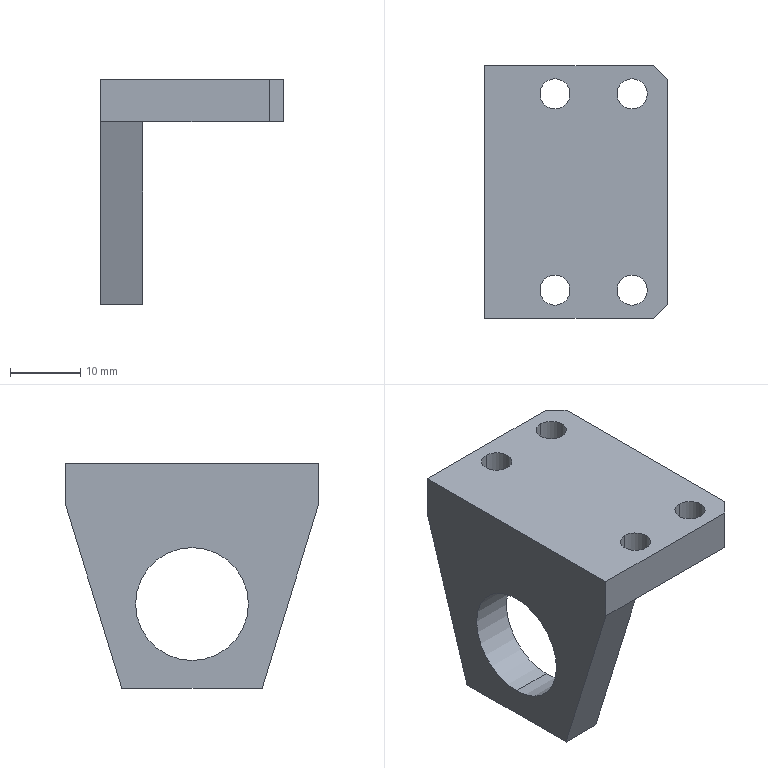Component | SolidWorks | 05-1111-1 | 1 solid | 22 faces | box 26 x 36 x 32 mm | volume 8390 mm3 | plane 12 | cylinder 10 | commonest cylinder face diameters 4.3 x8 16.1 x2 | material Plain Carbon Steel
build123d program:
from build123d import *

# Parameters (mm, degrees)
BOSS_EXTRUDE1_DEPTH        = 18
SKETCH2_R                  = 8.05
CUT_EXTRUDE1_DEPTH         = 42.809
F_4_3_4_3_DIAMETER_HOLE1_D = 4.3
CHAMFER1_SIZE              = 2
CUT_EXTRUDE4_DEPTH         = 41.939


with BuildPart() as part:
    # Sketch1 → Boss-Extrude1 (new, symmetric)
    with BuildSketch(Plane.XY):
        Polygon((0, 0), (32, 0), (32, 6), (6, 6), (6, 26), (0, 26), align=None)
    extrude(amount=BOSS_EXTRUDE1_DEPTH, both=True)

    # Sketch2 → Cut-Extrude1 (cut, through all)
    with BuildSketch(Plane(origin=(0, 6, 0), x_dir=(1, 0, 0), z_dir=(0, 1, 0))):
        with Locations(Location((20, 0, 0), (0, 0, 180))):
            Circle(SKETCH2_R)
    extrude(amount=-CUT_EXTRUDE1_DEPTH, mode=Mode.SUBTRACT)

    # 4.3 _4.3_ Diameter Hole1 (through all)
    with Locations(Plane(origin=(6, 0, 0), x_dir=(0, 0, -1), z_dir=(1, 0, 0))):
        with Locations((-14, 21), (-14, 10), (14, 10), (14, 21)):
            Hole(F_4_3_4_3_DIAMETER_HOLE1_D / 2)

    # Chamfer1
    chamfer1_edges = [part.edges().sort_by_distance(p)[0] for p in [
        (3, 26, 18),
        (3, 26, -18),
    ]]
    chamfer(chamfer1_edges, length=CHAMFER1_SIZE)

    # Sketch5 → Cut-Extrude4 (cut, through all)
    with BuildSketch(Plane(origin=(6, 0, 0), x_dir=(0, 0, -1), z_dir=(0, 1, 0))):
        Polygon((-18, -26), (-10, -26), (-18, 0), align=None)
        Polygon((10, -26), (18, 0), (18, -26), align=None)
    extrude(amount=CUT_EXTRUDE4_DEPTH, mode=Mode.SUBTRACT)


solid = part.part

# Placed as in the assembly
solid = solid.moved(Location((-105, 24, -6), (90, 0, -90)))
STEP:
#1=CARTESIAN_POINT('',(-3.307,0.3091,-0.2362));
#2=VERTEX_POINT('',#1);
#3=CARTESIAN_POINT('',(-3.307,0.4783,-0.2362));
#4=VERTEX_POINT('',#3);
#5=CARTESIAN_POINT('',(-3.307,0.3937,-0.2362));
#6=DIRECTION('',(0.,0.,-1.));
#7=DIRECTION('',(0.,1.,0.));
#8=AXIS2_PLACEMENT_3D('',#5,#6,#7);
#9=CIRCLE('',#8,0.08465);
#10=EDGE_CURVE('',#2,#4,#9,.T.);
#11=ORIENTED_EDGE('',*,*,#10,.F.);
#12=CARTESIAN_POINT('',(-3.307,0.3091,-0.4724));
#13=VERTEX_POINT('',#12);
#14=CARTESIAN_POINT('',(-3.307,0.3091,-0.4724));
#15=DIRECTION('',(0.,0.,-1.));
#16=VECTOR('',#15,39.37);
#17=LINE('',#14,#16);
#18=EDGE_CURVE('',#2,#13,#17,.T.);
#19=ORIENTED_EDGE('',*,*,#18,.T.);
#20=CARTESIAN_POINT('',(-3.307,0.4783,-0.4724));
#21=VERTEX_POINT('',#20);
#22=CARTESIAN_POINT('',(-3.307,0.3937,-0.4724));
#23=DIRECTION('',(0.,0.,-1.));
#24=DIRECTION('',(0.,1.,0.));
#25=AXIS2_PLACEMENT_3D('',#22,#23,#24);
#26=CIRCLE('',#25,0.08465);
#27=EDGE_CURVE('',#13,#21,#26,.T.);
#28=ORIENTED_EDGE('',*,*,#27,.T.);
#29=CARTESIAN_POINT('',(-3.307,0.4783,-0.4724));
#30=DIRECTION('',(0.,0.,-1.));
#31=VECTOR('',#30,39.37);
#32=LINE('',#29,#31);
#33=EDGE_CURVE('',#4,#21,#32,.T.);
#34=ORIENTED_EDGE('',*,*,#33,.F.);
#35=EDGE_LOOP('',(#11,#19,#28,#34));
#36=FACE_OUTER_BOUND('',#35,.T.);
#37=CARTESIAN_POINT('',(-3.307,0.3937,-0.4724));
#38=DIRECTION('',(0.,0.,-1.));
#39=DIRECTION('',(0.,1.,0.));
#40=AXIS2_PLACEMENT_3D('',#37,#38,#39);
#41=CYLINDRICAL_SURFACE('',#40,0.08465);
#42=ADVANCED_FACE('',(#36),#41,.F.);
#43=CARTESIAN_POINT('',(-3.74,0.3091,-0.2362));
#44=VERTEX_POINT('',#43);
#45=CARTESIAN_POINT('',(-3.74,0.4783,-0.2362));
#46=VERTEX_POINT('',#45);
#47=CARTESIAN_POINT('',(-3.74,0.3937,-0.2362));
#48=DIRECTION('',(0.,0.,-1.));
#49=DIRECTION('',(0.,1.,0.));
#50=AXIS2_PLACEMENT_3D('',#47,#48,#49);
#51=CIRCLE('',#50,0.08465);
#52=EDGE_CURVE('',#44,#46,#51,.T.);
#53=ORIENTED_EDGE('',*,*,#52,.F.);
#54=CARTESIAN_POINT('',(-3.74,0.3091,-0.4724));
#55=VERTEX_POINT('',#54);
#56=CARTESIAN_POINT('',(-3.74,0.3091,-0.4724));
#57=DIRECTION('',(0.,0.,-1.));
#58=VECTOR('',#57,39.37);
#59=LINE('',#56,#58);
#60=EDGE_CURVE('',#44,#55,#59,.T.);
#61=ORIENTED_EDGE('',*,*,#60,.T.);
#62=CARTESIAN_POINT('',(-3.74,0.4783,-0.4724));
#63=VERTEX_POINT('',#62);
#64=CARTESIAN_POINT('',(-3.74,0.3937,-0.4724));
#65=DIRECTION('',(0.,0.,-1.));
#66=DIRECTION('',(0.,1.,0.));
#67=AXIS2_PLACEMENT_3D('',#64,#65,#66);
#68=CIRCLE('',#67,0.08465);
#69=EDGE_CURVE('',#55,#63,#68,.T.);
#70=ORIENTED_EDGE('',*,*,#69,.T.);
#71=CARTESIAN_POINT('',(-3.74,0.4783,-0.4724));
#72=DIRECTION('',(0.,0.,-1.));
#73=VECTOR('',#72,39.37);
#74=LINE('',#71,#73);
#75=EDGE_CURVE('',#46,#63,#74,.T.);
#76=ORIENTED_EDGE('',*,*,#75,.F.);
#77=EDGE_LOOP('',(#53,#61,#70,#76));
#78=FACE_OUTER_BOUND('',#77,.T.);
#79=CARTESIAN_POINT('',(-3.74,0.3937,-0.4724));
#80=DIRECTION('',(0.,0.,-1.));
#81=DIRECTION('',(0.,1.,0.));
#82=AXIS2_PLACEMENT_3D('',#79,#80,#81);
#83=CYLINDRICAL_SURFACE('',#82,0.08465);
#84=ADVANCED_FACE('',(#78),#83,.F.);
#85=CARTESIAN_POINT('',(-3.74,1.411,-0.2362));
#86=VERTEX_POINT('',#85);
#87=CARTESIAN_POINT('',(-3.74,1.581,-0.2362));
#88=VERTEX_POINT('',#87);
#89=CARTESIAN_POINT('',(-3.74,1.496,-0.2362));
#90=DIRECTION('',(0.,0.,-1.));
#91=DIRECTION('',(0.,1.,0.));
#92=AXIS2_PLACEMENT_3D('',#89,#90,#91);
#93=CIRCLE('',#92,0.08465);
#94=EDGE_CURVE('',#86,#88,#93,.T.);
#95=ORIENTED_EDGE('',*,*,#94,.F.);
#96=CARTESIAN_POINT('',(-3.74,1.411,-0.4724));
#97=VERTEX_POINT('',#96);
#98=CARTESIAN_POINT('',(-3.74,1.411,-0.4724));
#99=DIRECTION('',(0.,0.,-1.));
#100=VECTOR('',#99,39.37);
#101=LINE('',#98,#100);
#102=EDGE_CURVE('',#86,#97,#101,.T.);
#103=ORIENTED_EDGE('',*,*,#102,.T.);
#104=CARTESIAN_POINT('',(-3.74,1.581,-0.4724));
#105=VERTEX_POINT('',#104);
#106=CARTESIAN_POINT('',(-3.74,1.496,-0.4724));
#107=DIRECTION('',(0.,0.,-1.));
#108=DIRECTION('',(0.,1.,0.));
#109=AXIS2_PLACEMENT_3D('',#106,#107,#108);
#110=CIRCLE('',#109,0.08465);
#111=EDGE_CURVE('',#97,#105,#110,.T.);
#112=ORIENTED_EDGE('',*,*,#111,.T.);
#113=CARTESIAN_POINT('',(-3.74,1.581,-0.4724));
#114=DIRECTION('',(0.,0.,-1.));
#115=VECTOR('',#114,39.37);
#116=LINE('',#113,#115);
#117=EDGE_CURVE('',#88,#105,#116,.T.);
#118=ORIENTED_EDGE('',*,*,#117,.F.);
#119=EDGE_LOOP('',(#95,#103,#112,#118));
#120=FACE_OUTER_BOUND('',#119,.T.);
#121=CARTESIAN_POINT('',(-3.74,1.496,-0.4724));
#122=DIRECTION('',(0.,0.,-1.));
#123=DIRECTION('',(0.,1.,0.));
#124=AXIS2_PLACEMENT_3D('',#121,#122,#123);
#125=CYLINDRICAL_SURFACE('',#124,0.08465);
#126=ADVANCED_FACE('',(#120),#125,.F.);
#127=CARTESIAN_POINT('',(-3.307,1.411,-0.2362));
#128=VERTEX_POINT('',#127);
#129=CARTESIAN_POINT('',(-3.307,1.581,-0.2362));
#130=VERTEX_POINT('',#129);
#131=CARTESIAN_POINT('',(-3.307,1.496,-0.2362));
#132=DIRECTION('',(0.,0.,-1.));
#133=DIRECTION('',(0.,1.,0.));
#134=AXIS2_PLACEMENT_3D('',#131,#132,#133);
#135=CIRCLE('',#134,0.08465);
#136=EDGE_CURVE('',#128,#130,#135,.T.);
#137=ORIENTED_EDGE('',*,*,#136,.F.);
#138=CARTESIAN_POINT('',(-3.307,1.411,-0.4724));
#139=VERTEX_POINT('',#138);
#140=CARTESIAN_POINT('',(-3.307,1.411,-0.4724));
#141=DIRECTION('',(0.,0.,-1.));
#142=VECTOR('',#141,39.37);
#143=LINE('',#140,#142);
#144=EDGE_CURVE('',#128,#139,#143,.T.);
#145=ORIENTED_EDGE('',*,*,#144,.T.);
#146=CARTESIAN_POINT('',(-3.307,1.581,-0.4724));
#147=VERTEX_POINT('',#146);
#148=CARTESIAN_POINT('',(-3.307,1.496,-0.4724));
#149=DIRECTION('',(0.,0.,-1.));
#150=DIRECTION('',(0.,1.,0.));
#151=AXIS2_PLACEMENT_3D('',#148,#149,#150);
#152=CIRCLE('',#151,0.08465);
#153=EDGE_CURVE('',#139,#147,#152,.T.);
#154=ORIENTED_EDGE('',*,*,#153,.T.);
#155=CARTESIAN_POINT('',(-3.307,1.581,-0.4724));
#156=DIRECTION('',(0.,0.,-1.));
#157=VECTOR('',#156,39.37);
#158=LINE('',#155,#157);
#159=EDGE_CURVE('',#130,#147,#158,.T.);
#160=ORIENTED_EDGE('',*,*,#159,.F.);
#161=EDGE_LOOP('',(#137,#145,#154,#160));
#162=FACE_OUTER_BOUND('',#161,.T.);
#163=CARTESIAN_POINT('',(-3.307,1.496,-0.4724));
#164=DIRECTION('',(0.,0.,-1.));
#165=DIRECTION('',(0.,1.,0.));
#166=AXIS2_PLACEMENT_3D('',#163,#164,#165);
#167=CYLINDRICAL_SURFACE('',#166,0.08465);
#168=ADVANCED_FACE('',(#162),#167,.F.);
#169=CARTESIAN_POINT('',(-4.134,0.9449,-1.341));
#170=VERTEX_POINT('',#169);
#171=CARTESIAN_POINT('',(-4.134,0.9449,-0.7067));
#172=VERTEX_POINT('',#171);
#173=CARTESIAN_POINT('',(-4.134,0.9449,-1.024));
#174=DIRECTION('',(1.,0.,-0.));
#175=DIRECTION('',(0.,0.,1.));
#176=AXIS2_PLACEMENT_3D('',#173,#174,#175);
#177=CIRCLE('',#176,0.3169);
#178=EDGE_CURVE('',#170,#172,#177,.T.);
#179=ORIENTED_EDGE('',*,*,#178,.F.);
#180=CARTESIAN_POINT('',(-3.898,0.9449,-1.341));
#181=VERTEX_POINT('',#180);
#182=CARTESIAN_POINT('',(-4.134,0.9449,-1.341));
#183=DIRECTION('',(1.,0.,-0.));
#184=VECTOR('',#183,39.37);
#185=LINE('',#182,#184);
#186=EDGE_CURVE('',#170,#181,#185,.T.);
#187=ORIENTED_EDGE('',*,*,#186,.T.);
#188=CARTESIAN_POINT('',(-3.898,0.9449,-0.7067));
#189=VERTEX_POINT('',#188);
#190=CARTESIAN_POINT('',(-3.898,0.9449,-1.024));
#191=DIRECTION('',(1.,0.,-0.));
#192=DIRECTION('',(0.,0.,1.));
#193=AXIS2_PLACEMENT_3D('',#190,#191,#192);
#194=CIRCLE('',#193,0.3169);
#195=EDGE_CURVE('',#181,#189,#194,.T.);
#196=ORIENTED_EDGE('',*,*,#195,.T.);
#197=CARTESIAN_POINT('',(-4.134,0.9449,-0.7067));
#198=DIRECTION('',(1.,0.,-0.));
#199=VECTOR('',#198,39.37);
#200=LINE('',#197,#199);
#201=EDGE_CURVE('',#172,#189,#200,.T.);
#202=ORIENTED_EDGE('',*,*,#201,.F.);
#203=EDGE_LOOP('',(#179,#187,#196,#202));
#204=FACE_OUTER_BOUND('',#203,.T.);
#205=CARTESIAN_POINT('',(-4.134,0.9449,-1.024));
#206=DIRECTION('',(1.,0.,-0.));
#207=DIRECTION('',(0.,0.,1.));
#208=AXIS2_PLACEMENT_3D('',#205,#206,#207);
#209=CYLINDRICAL_SURFACE('',#208,0.3169);
#210=ADVANCED_FACE('',(#204),#209,.F.);
#211=CARTESIAN_POINT('',(-4.134,0.9449,-1.024));
#212=DIRECTION('',(1.,0.,-0.));
#213=DIRECTION('',(0.,0.,1.));
#214=AXIS2_PLACEMENT_3D('',#211,#212,#213);
#215=CIRCLE('',#214,0.3169);
#216=EDGE_CURVE('',#172,#170,#215,.T.);
#217=ORIENTED_EDGE('',*,*,#216,.T.);
#218=ORIENTED_EDGE('',*,*,#178,.T.);
#219=EDGE_LOOP('',(#217,#218));
#220=FACE_BOUND('',#219,.T.);
#221=CARTESIAN_POINT('',(-4.134,1.654,-0.4724));
#222=VERTEX_POINT('',#221);
#223=CARTESIAN_POINT('',(-4.134,1.339,-1.496));
#224=VERTEX_POINT('',#223);
#225=CARTESIAN_POINT('',(-4.134,1.339,-1.496));
#226=DIRECTION('',(0.,-0.2941,-0.9558));
#227=VECTOR('',#226,39.37);
#228=LINE('',#225,#227);
#229=EDGE_CURVE('',#222,#224,#228,.T.);
#230=ORIENTED_EDGE('',*,*,#229,.T.);
#231=CARTESIAN_POINT('',(-4.134,0.5512,-1.496));
#232=VERTEX_POINT('',#231);
#233=CARTESIAN_POINT('',(-4.134,0.2362,-1.496));
#234=DIRECTION('',(0.,1.,0.));
#235=VECTOR('',#234,39.37);
#236=LINE('',#233,#235);
#237=EDGE_CURVE('',#232,#224,#236,.T.);
#238=ORIENTED_EDGE('',*,*,#237,.F.);
#239=CARTESIAN_POINT('',(-4.134,0.2362,-0.4724));
#240=VERTEX_POINT('',#239);
#241=CARTESIAN_POINT('',(-4.134,0.5512,-1.496));
#242=DIRECTION('',(-0.,-0.2941,0.9558));
#243=VECTOR('',#242,39.37);
#244=LINE('',#241,#243);
#245=EDGE_CURVE('',#232,#240,#244,.T.);
#246=ORIENTED_EDGE('',*,*,#245,.T.);
#247=CARTESIAN_POINT('',(-4.134,0.2362,-0.2362));
#248=VERTEX_POINT('',#247);
#249=CARTESIAN_POINT('',(-4.134,0.2362,-0.2362));
#250=DIRECTION('',(0.,0.,-1.));
#251=VECTOR('',#250,39.37);
#252=LINE('',#249,#251);
#253=EDGE_CURVE('',#248,#240,#252,.T.);
#254=ORIENTED_EDGE('',*,*,#253,.F.);
#255=CARTESIAN_POINT('',(-4.134,1.654,-0.2362));
#256=VERTEX_POINT('',#255);
#257=CARTESIAN_POINT('',(-4.134,0.2362,-0.2362));
#258=DIRECTION('',(0.,1.,0.));
#259=VECTOR('',#258,39.37);
#260=LINE('',#257,#259);
#261=EDGE_CURVE('',#248,#256,#260,.T.);
#262=ORIENTED_EDGE('',*,*,#261,.T.);
#263=CARTESIAN_POINT('',(-4.134,1.654,-0.2362));
#264=DIRECTION('',(0.,0.,-1.));
#265=VECTOR('',#264,39.37);
#266=LINE('',#263,#265);
#267=EDGE_CURVE('',#256,#222,#266,.T.);
#268=ORIENTED_EDGE('',*,*,#267,.T.);
#269=EDGE_LOOP('',(#230,#238,#246,#254,#262,#268));
#270=FACE_OUTER_BOUND('',#269,.T.);
#271=CARTESIAN_POINT('',(-4.134,0.2362,-0.2362));
#272=DIRECTION('',(1.,-0.,-0.));
#273=DIRECTION('',(-0.,-1.,-0.));
#274=AXIS2_PLACEMENT_3D('',#271,#272,#273);
#275=PLANE('',#274);
#276=ADVANCED_FACE('',(#220,#270),#275,.F.);
#277=CARTESIAN_POINT('',(-3.898,1.339,-1.496));
#278=VERTEX_POINT('',#277);
#279=CARTESIAN_POINT('',(-3.11,1.339,-1.496));
#280=DIRECTION('',(-1.,-0.,0.));
#281=VECTOR('',#280,39.37);
#282=LINE('',#279,#281);
#283=EDGE_CURVE('',#278,#224,#282,.T.);
#284=ORIENTED_EDGE('',*,*,#283,.F.);
#285=CARTESIAN_POINT('',(-3.898,0.5512,-1.496));
#286=VERTEX_POINT('',#285);
#287=CARTESIAN_POINT('',(-3.898,0.2362,-1.496));
#288=DIRECTION('',(0.,1.,0.));
#289=VECTOR('',#288,39.37);
#290=LINE('',#287,#289);
#291=EDGE_CURVE('',#286,#278,#290,.T.);
#292=ORIENTED_EDGE('',*,*,#291,.F.);
#293=CARTESIAN_POINT('',(-3.11,0.5512,-1.496));
#294=DIRECTION('',(-1.,-0.,0.));
#295=VECTOR('',#294,39.37);
#296=LINE('',#293,#295);
#297=EDGE_CURVE('',#286,#232,#296,.T.);
#298=ORIENTED_EDGE('',*,*,#297,.T.);
#299=ORIENTED_EDGE('',*,*,#237,.T.);
#300=EDGE_LOOP('',(#284,#292,#298,#299));
#301=FACE_OUTER_BOUND('',#300,.T.);
#302=CARTESIAN_POINT('',(-4.134,0.2362,-1.496));
#303=DIRECTION('',(-0.,-0.,1.));
#304=DIRECTION('',(-0.,-1.,-0.));
#305=AXIS2_PLACEMENT_3D('',#302,#303,#304);
#306=PLANE('',#305);
#307=ADVANCED_FACE('',(#301),#306,.F.);
#308=CARTESIAN_POINT('',(-3.898,0.9449,-1.024));
#309=DIRECTION('',(1.,0.,-0.));
#310=DIRECTION('',(0.,0.,1.));
#311=AXIS2_PLACEMENT_3D('',#308,#309,#310);
#312=CIRCLE('',#311,0.3169);
#313=EDGE_CURVE('',#189,#181,#312,.T.);
#314=ORIENTED_EDGE('',*,*,#313,.F.);
#315=ORIENTED_EDGE('',*,*,#195,.F.);
#316=EDGE_LOOP('',(#314,#315));
#317=FACE_BOUND('',#316,.T.);
#318=CARTESIAN_POINT('',(-3.898,1.654,-0.4724));
#319=VERTEX_POINT('',#318);
#320=CARTESIAN_POINT('',(-3.898,1.243,-1.806));
#321=DIRECTION('',(0.,-0.2941,-0.9558));
#322=VECTOR('',#321,39.37);
#323=LINE('',#320,#322);
#324=EDGE_CURVE('',#319,#278,#323,.T.);
#325=ORIENTED_EDGE('',*,*,#324,.F.);
#326=CARTESIAN_POINT('',(-3.898,0.2362,-0.4724));
#327=VERTEX_POINT('',#326);
#328=CARTESIAN_POINT('',(-3.898,0.2362,-0.4724));
#329=DIRECTION('',(0.,1.,0.));
#330=VECTOR('',#329,39.37);
#331=LINE('',#328,#330);
#332=EDGE_CURVE('',#327,#319,#331,.T.);
#333=ORIENTED_EDGE('',*,*,#332,.F.);
#334=CARTESIAN_POINT('',(-3.898,0.5239,-1.408));
#335=DIRECTION('',(-0.,-0.2941,0.9558));
#336=VECTOR('',#335,39.37);
#337=LINE('',#334,#336);
#338=EDGE_CURVE('',#286,#327,#337,.T.);
#339=ORIENTED_EDGE('',*,*,#338,.F.);
#340=ORIENTED_EDGE('',*,*,#291,.T.);
#341=EDGE_LOOP('',(#325,#333,#339,#340));
#342=FACE_OUTER_BOUND('',#341,.T.);
#343=CARTESIAN_POINT('',(-3.898,0.2362,-1.496));
#344=DIRECTION('',(-1.,-0.,-0.));
#345=DIRECTION('',(0.,0.,-1.));
#346=AXIS2_PLACEMENT_3D('',#343,#344,#345);
#347=PLANE('',#346);
#348=ADVANCED_FACE('',(#317,#342),#347,.F.);
#349=CARTESIAN_POINT('',(-4.134,1.654,-0.4724));
#350=DIRECTION('',(1.,0.,-0.));
#351=VECTOR('',#350,39.37);
#352=LINE('',#349,#351);
#353=EDGE_CURVE('',#222,#319,#352,.T.);
#354=ORIENTED_EDGE('',*,*,#353,.F.);
#355=ORIENTED_EDGE('',*,*,#267,.F.);
#356=CARTESIAN_POINT('',(-3.189,1.654,-0.2362));
#357=VERTEX_POINT('',#356);
#358=CARTESIAN_POINT('',(-3.11,1.654,-0.2362));
#359=DIRECTION('',(-1.,-0.,0.));
#360=VECTOR('',#359,39.37);
#361=LINE('',#358,#360);
#362=EDGE_CURVE('',#357,#256,#361,.T.);
#363=ORIENTED_EDGE('',*,*,#362,.F.);
#364=CARTESIAN_POINT('',(-3.189,1.654,-0.4724));
#365=VERTEX_POINT('',#364);
#366=CARTESIAN_POINT('',(-3.189,1.654,-0.2362));
#367=DIRECTION('',(0.,0.,-1.));
#368=VECTOR('',#367,39.37);
#369=LINE('',#366,#368);
#370=EDGE_CURVE('',#357,#365,#369,.T.);
#371=ORIENTED_EDGE('',*,*,#370,.T.);
#372=CARTESIAN_POINT('',(-3.898,1.654,-0.4724));
#373=DIRECTION('',(1.,0.,-0.));
#374=VECTOR('',#373,39.37);
#375=LINE('',#372,#374);
#376=EDGE_CURVE('',#319,#365,#375,.T.);
#377=ORIENTED_EDGE('',*,*,#376,.F.);
#378=EDGE_LOOP('',(#354,#355,#363,#371,#377));
#379=FACE_OUTER_BOUND('',#378,.T.);
#380=CARTESIAN_POINT('',(-4.134,1.654,-0.2362));
#381=DIRECTION('',(-0.,-1.,-0.));
#382=DIRECTION('',(0.,0.,-1.));
#383=AXIS2_PLACEMENT_3D('',#380,#381,#382);
#384=PLANE('',#383);
#385=ADVANCED_FACE('',(#379),#384,.F.);
#386=ORIENTED_EDGE('',*,*,#253,.T.);
#387=CARTESIAN_POINT('',(-4.134,0.2362,-0.4724));
#388=DIRECTION('',(1.,0.,-0.));
#389=VECTOR('',#388,39.37);
#390=LINE('',#387,#389);
#391=EDGE_CURVE('',#240,#327,#390,.T.);
#392=ORIENTED_EDGE('',*,*,#391,.T.);
#393=CARTESIAN_POINT('',(-3.189,0.2362,-0.4724));
#394=VERTEX_POINT('',#393);
#395=CARTESIAN_POINT('',(-3.898,0.2362,-0.4724));
#396=DIRECTION('',(1.,0.,-0.));
#397=VECTOR('',#396,39.37);
#398=LINE('',#395,#397);
#399=EDGE_CURVE('',#327,#394,#398,.T.);
#400=ORIENTED_EDGE('',*,*,#399,.T.);
#401=CARTESIAN_POINT('',(-3.189,0.2362,-0.2362));
#402=VERTEX_POINT('',#401);
#403=CARTESIAN_POINT('',(-3.189,0.2362,-0.2362));
#404=DIRECTION('',(-0.,-0.,1.));
#405=VECTOR('',#404,39.37);
#406=LINE('',#403,#405);
#407=EDGE_CURVE('',#394,#402,#406,.T.);
#408=ORIENTED_EDGE('',*,*,#407,.T.);
#409=CARTESIAN_POINT('',(-3.11,0.2362,-0.2362));
#410=DIRECTION('',(-1.,-0.,0.));
#411=VECTOR('',#410,39.37);
#412=LINE('',#409,#411);
#413=EDGE_CURVE('',#402,#248,#412,.T.);
#414=ORIENTED_EDGE('',*,*,#413,.T.);
#415=EDGE_LOOP('',(#386,#392,#400,#408,#414));
#416=FACE_OUTER_BOUND('',#415,.T.);
#417=CARTESIAN_POINT('',(-4.134,0.2362,-0.2362));
#418=DIRECTION('',(-0.,-1.,-0.));
#419=DIRECTION('',(0.,0.,-1.));
#420=AXIS2_PLACEMENT_3D('',#417,#418,#419);
#421=PLANE('',#420);
#422=ADVANCED_FACE('',(#416),#421,.T.);
#423=CARTESIAN_POINT('',(-3.307,0.3937,-0.2362));
#424=DIRECTION('',(0.,0.,-1.));
#425=DIRECTION('',(0.,1.,0.));
#426=AXIS2_PLACEMENT_3D('',#423,#424,#425);
#427=CIRCLE('',#426,0.08465);
#428=EDGE_CURVE('',#4,#2,#427,.T.);
#429=ORIENTED_EDGE('',*,*,#428,.T.);
#430=ORIENTED_EDGE('',*,*,#10,.T.);
#431=EDGE_LOOP('',(#429,#430));
#432=FACE_BOUND('',#431,.T.);
#433=CARTESIAN_POINT('',(-3.74,0.3937,-0.2362));
#434=DIRECTION('',(0.,0.,-1.));
#435=DIRECTION('',(0.,1.,0.));
#436=AXIS2_PLACEMENT_3D('',#433,#434,#435);
#437=CIRCLE('',#436,0.08465);
#438=EDGE_CURVE('',#46,#44,#437,.T.);
#439=ORIENTED_EDGE('',*,*,#438,.T.);
#440=ORIENTED_EDGE('',*,*,#52,.T.);
#441=EDGE_LOOP('',(#439,#440));
#442=FACE_BOUND('',#441,.T.);
#443=CARTESIAN_POINT('',(-3.74,1.496,-0.2362));
#444=DIRECTION('',(0.,0.,-1.));
#445=DIRECTION('',(0.,1.,0.));
#446=AXIS2_PLACEMENT_3D('',#443,#444,#445);
#447=CIRCLE('',#446,0.08465);
#448=EDGE_CURVE('',#88,#86,#447,.T.);
#449=ORIENTED_EDGE('',*,*,#448,.T.);
#450=ORIENTED_EDGE('',*,*,#94,.T.);
#451=EDGE_LOOP('',(#449,#450));
#452=FACE_BOUND('',#451,.T.);
#453=CARTESIAN_POINT('',(-3.307,1.496,-0.2362));
#454=DIRECTION('',(0.,0.,-1.));
#455=DIRECTION('',(0.,1.,0.));
#456=AXIS2_PLACEMENT_3D('',#453,#454,#455);
#457=CIRCLE('',#456,0.08465);
#458=EDGE_CURVE('',#130,#128,#457,.T.);
#459=ORIENTED_EDGE('',*,*,#458,.T.);
#460=ORIENTED_EDGE('',*,*,#136,.T.);
#461=EDGE_LOOP('',(#459,#460));
#462=FACE_BOUND('',#461,.T.);
#463=CARTESIAN_POINT('',(-3.11,0.315,-0.2362));
#464=VERTEX_POINT('',#463);
#465=CARTESIAN_POINT('',(-3.11,1.575,-0.2362));
#466=VERTEX_POINT('',#465);
#467=CARTESIAN_POINT('',(-3.11,0.2362,-0.2362));
#468=DIRECTION('',(0.,1.,0.));
#469=VECTOR('',#468,39.37);
#470=LINE('',#467,#469);
#471=EDGE_CURVE('',#464,#466,#470,.T.);
#472=ORIENTED_EDGE('',*,*,#471,.T.);
#473=CARTESIAN_POINT('',(-3.11,1.575,-0.2362));
#474=DIRECTION('',(-0.7071,0.7071,0.));
#475=VECTOR('',#474,39.37);
#476=LINE('',#473,#475);
#477=EDGE_CURVE('',#466,#357,#476,.T.);
#478=ORIENTED_EDGE('',*,*,#477,.T.);
#479=ORIENTED_EDGE('',*,*,#362,.T.);
#480=ORIENTED_EDGE('',*,*,#261,.F.);
#481=ORIENTED_EDGE('',*,*,#413,.F.);
#482=CARTESIAN_POINT('',(-3.189,0.2362,-0.2362));
#483=DIRECTION('',(0.7071,0.7071,-0.));
#484=VECTOR('',#483,39.37);
#485=LINE('',#482,#484);
#486=EDGE_CURVE('',#402,#464,#485,.T.);
#487=ORIENTED_EDGE('',*,*,#486,.T.);
#488=EDGE_LOOP('',(#472,#478,#479,#480,#481,#487));
#489=FACE_OUTER_BOUND('',#488,.T.);
#490=CARTESIAN_POINT('',(-3.11,0.2362,-0.2362));
#491=DIRECTION('',(-0.,0.,-1.));
#492=DIRECTION('',(1.,0.,-0.));
#493=AXIS2_PLACEMENT_3D('',#490,#491,#492);
#494=PLANE('',#493);
#495=ADVANCED_FACE('',(#432,#442,#452,#462,#489),#494,.F.);
#496=CARTESIAN_POINT('',(-3.307,0.3937,-0.4724));
#497=DIRECTION('',(0.,0.,-1.));
#498=DIRECTION('',(0.,1.,0.));
#499=AXIS2_PLACEMENT_3D('',#496,#497,#498);
#500=CIRCLE('',#499,0.08465);
#501=EDGE_CURVE('',#21,#13,#500,.T.);
#502=ORIENTED_EDGE('',*,*,#501,.F.);
#503=ORIENTED_EDGE('',*,*,#27,.F.);
#504=EDGE_LOOP('',(#502,#503));
#505=FACE_BOUND('',#504,.T.);
#506=CARTESIAN_POINT('',(-3.74,0.3937,-0.4724));
#507=DIRECTION('',(0.,0.,-1.));
#508=DIRECTION('',(0.,1.,0.));
#509=AXIS2_PLACEMENT_3D('',#506,#507,#508);
#510=CIRCLE('',#509,0.08465);
#511=EDGE_CURVE('',#63,#55,#510,.T.);
#512=ORIENTED_EDGE('',*,*,#511,.F.);
#513=ORIENTED_EDGE('',*,*,#69,.F.);
#514=EDGE_LOOP('',(#512,#513));
#515=FACE_BOUND('',#514,.T.);
#516=CARTESIAN_POINT('',(-3.74,1.496,-0.4724));
#517=DIRECTION('',(0.,0.,-1.));
#518=DIRECTION('',(0.,1.,0.));
#519=AXIS2_PLACEMENT_3D('',#516,#517,#518);
#520=CIRCLE('',#519,0.08465);
#521=EDGE_CURVE('',#105,#97,#520,.T.);
#522=ORIENTED_EDGE('',*,*,#521,.F.);
#523=ORIENTED_EDGE('',*,*,#111,.F.);
#524=EDGE_LOOP('',(#522,#523));
#525=FACE_BOUND('',#524,.T.);
#526=CARTESIAN_POINT('',(-3.307,1.496,-0.4724));
#527=DIRECTION('',(0.,0.,-1.));
#528=DIRECTION('',(0.,1.,0.));
#529=AXIS2_PLACEMENT_3D('',#526,#527,#528);
#530=CIRCLE('',#529,0.08465);
#531=EDGE_CURVE('',#147,#139,#530,.T.);
#532=ORIENTED_EDGE('',*,*,#531,.F.);
#533=ORIENTED_EDGE('',*,*,#153,.F.);
#534=EDGE_LOOP('',(#532,#533));
#535=FACE_BOUND('',#534,.T.);
#536=ORIENTED_EDGE('',*,*,#376,.T.);
#537=CARTESIAN_POINT('',(-3.11,1.575,-0.4724));
#538=VERTEX_POINT('',#537);
#539=CARTESIAN_POINT('',(-3.11,1.575,-0.4724));
#540=DIRECTION('',(0.7071,-0.7071,-0.));
#541=VECTOR('',#540,39.37);
#542=LINE('',#539,#541);
#543=EDGE_CURVE('',#365,#538,#542,.T.);
#544=ORIENTED_EDGE('',*,*,#543,.T.);
#545=CARTESIAN_POINT('',(-3.11,0.315,-0.4724));
#546=VERTEX_POINT('',#545);
#547=CARTESIAN_POINT('',(-3.11,0.2362,-0.4724));
#548=DIRECTION('',(0.,1.,0.));
#549=VECTOR('',#548,39.37);
#550=LINE('',#547,#549);
#551=EDGE_CURVE('',#546,#538,#550,.T.);
#552=ORIENTED_EDGE('',*,*,#551,.F.);
#553=CARTESIAN_POINT('',(-3.189,0.2362,-0.4724));
#554=DIRECTION('',(-0.7071,-0.7071,0.));
#555=VECTOR('',#554,39.37);
#556=LINE('',#553,#555);
#557=EDGE_CURVE('',#546,#394,#556,.T.);
#558=ORIENTED_EDGE('',*,*,#557,.T.);
#559=ORIENTED_EDGE('',*,*,#399,.F.);
#560=ORIENTED_EDGE('',*,*,#332,.T.);
#561=EDGE_LOOP('',(#536,#544,#552,#558,#559,#560));
#562=FACE_OUTER_BOUND('',#561,.T.);
#563=CARTESIAN_POINT('',(-3.898,0.2362,-0.4724));
#564=DIRECTION('',(0.,-0.,1.));
#565=DIRECTION('',(-1.,-0.,0.));
#566=AXIS2_PLACEMENT_3D('',#563,#564,#565);
#567=PLANE('',#566);
#568=ADVANCED_FACE('',(#505,#515,#525,#535,#562),#567,.F.);
#569=ORIENTED_EDGE('',*,*,#551,.T.);
#570=CARTESIAN_POINT('',(-3.11,1.575,-0.4724));
#571=DIRECTION('',(-0.,-0.,1.));
#572=VECTOR('',#571,39.37);
#573=LINE('',#570,#572);
#574=EDGE_CURVE('',#538,#466,#573,.T.);
#575=ORIENTED_EDGE('',*,*,#574,.T.);
#576=ORIENTED_EDGE('',*,*,#471,.F.);
#577=CARTESIAN_POINT('',(-3.11,0.315,-0.4724));
#578=DIRECTION('',(0.,0.,-1.));
#579=VECTOR('',#578,39.37);
#580=LINE('',#577,#579);
#581=EDGE_CURVE('',#464,#546,#580,.T.);
#582=ORIENTED_EDGE('',*,*,#581,.T.);
#583=EDGE_LOOP('',(#569,#575,#576,#582));
#584=FACE_OUTER_BOUND('',#583,.T.);
#585=CARTESIAN_POINT('',(-3.11,0.2362,-0.4724));
#586=DIRECTION('',(-1.,0.,0.));
#587=DIRECTION('',(0.,1.,0.));
#588=AXIS2_PLACEMENT_3D('',#585,#586,#587);
#589=PLANE('',#588);
#590=ADVANCED_FACE('',(#584),#589,.F.);
#591=ORIENTED_EDGE('',*,*,#186,.F.);
#592=ORIENTED_EDGE('',*,*,#216,.F.);
#593=ORIENTED_EDGE('',*,*,#201,.T.);
#594=ORIENTED_EDGE('',*,*,#313,.T.);
#595=EDGE_LOOP('',(#591,#592,#593,#594));
#596=FACE_OUTER_BOUND('',#595,.T.);
#597=CARTESIAN_POINT('',(-4.134,0.9449,-1.024));
#598=DIRECTION('',(1.,0.,-0.));
#599=DIRECTION('',(0.,0.,1.));
#600=AXIS2_PLACEMENT_3D('',#597,#598,#599);
#601=CYLINDRICAL_SURFACE('',#600,0.3169);
#602=ADVANCED_FACE('',(#596),#601,.F.);
#603=ORIENTED_EDGE('',*,*,#144,.F.);
#604=ORIENTED_EDGE('',*,*,#458,.F.);
#605=ORIENTED_EDGE('',*,*,#159,.T.);
#606=ORIENTED_EDGE('',*,*,#531,.T.);
#607=EDGE_LOOP('',(#603,#604,#605,#606));
#608=FACE_OUTER_BOUND('',#607,.T.);
#609=CARTESIAN_POINT('',(-3.307,1.496,-0.4724));
#610=DIRECTION('',(0.,0.,-1.));
#611=DIRECTION('',(0.,1.,0.));
#612=AXIS2_PLACEMENT_3D('',#609,#610,#611);
#613=CYLINDRICAL_SURFACE('',#612,0.08465);
#614=ADVANCED_FACE('',(#608),#613,.F.);
#615=ORIENTED_EDGE('',*,*,#102,.F.);
#616=ORIENTED_EDGE('',*,*,#448,.F.);
#617=ORIENTED_EDGE('',*,*,#117,.T.);
#618=ORIENTED_EDGE('',*,*,#521,.T.);
#619=EDGE_LOOP('',(#615,#616,#617,#618));
#620=FACE_OUTER_BOUND('',#619,.T.);
#621=CARTESIAN_POINT('',(-3.74,1.496,-0.4724));
#622=DIRECTION('',(0.,0.,-1.));
#623=DIRECTION('',(0.,1.,0.));
#624=AXIS2_PLACEMENT_3D('',#621,#622,#623);
#625=CYLINDRICAL_SURFACE('',#624,0.08465);
#626=ADVANCED_FACE('',(#620),#625,.F.);
#627=ORIENTED_EDGE('',*,*,#60,.F.);
#628=ORIENTED_EDGE('',*,*,#438,.F.);
#629=ORIENTED_EDGE('',*,*,#75,.T.);
#630=ORIENTED_EDGE('',*,*,#511,.T.);
#631=EDGE_LOOP('',(#627,#628,#629,#630));
#632=FACE_OUTER_BOUND('',#631,.T.);
#633=CARTESIAN_POINT('',(-3.74,0.3937,-0.4724));
#634=DIRECTION('',(0.,0.,-1.));
#635=DIRECTION('',(0.,1.,0.));
#636=AXIS2_PLACEMENT_3D('',#633,#634,#635);
#637=CYLINDRICAL_SURFACE('',#636,0.08465);
#638=ADVANCED_FACE('',(#632),#637,.F.);
#639=ORIENTED_EDGE('',*,*,#18,.F.);
#640=ORIENTED_EDGE('',*,*,#428,.F.);
#641=ORIENTED_EDGE('',*,*,#33,.T.);
#642=ORIENTED_EDGE('',*,*,#501,.T.);
#643=EDGE_LOOP('',(#639,#640,#641,#642));
#644=FACE_OUTER_BOUND('',#643,.T.);
#645=CARTESIAN_POINT('',(-3.307,0.3937,-0.4724));
#646=DIRECTION('',(0.,0.,-1.));
#647=DIRECTION('',(0.,1.,0.));
#648=AXIS2_PLACEMENT_3D('',#645,#646,#647);
#649=CYLINDRICAL_SURFACE('',#648,0.08465);
#650=ADVANCED_FACE('',(#644),#649,.F.);
#651=ORIENTED_EDGE('',*,*,#543,.F.);
#652=ORIENTED_EDGE('',*,*,#370,.F.);
#653=ORIENTED_EDGE('',*,*,#477,.F.);
#654=ORIENTED_EDGE('',*,*,#574,.F.);
#655=EDGE_LOOP('',(#651,#652,#653,#654));
#656=FACE_OUTER_BOUND('',#655,.T.);
#657=CARTESIAN_POINT('',(-3.11,1.575,-0.4724));
#658=DIRECTION('',(-0.7071,-0.7071,-0.));
#659=DIRECTION('',(-0.,-0.,1.));
#660=AXIS2_PLACEMENT_3D('',#657,#658,#659);
#661=PLANE('',#660);
#662=ADVANCED_FACE('',(#656),#661,.F.);
#663=ORIENTED_EDGE('',*,*,#557,.F.);
#664=ORIENTED_EDGE('',*,*,#581,.F.);
#665=ORIENTED_EDGE('',*,*,#486,.F.);
#666=ORIENTED_EDGE('',*,*,#407,.F.);
#667=EDGE_LOOP('',(#663,#664,#665,#666));
#668=FACE_OUTER_BOUND('',#667,.T.);
#669=CARTESIAN_POINT('',(-3.189,0.2362,-0.2362));
#670=DIRECTION('',(0.7071,-0.7071,0.));
#671=DIRECTION('',(0.,0.,-1.));
#672=AXIS2_PLACEMENT_3D('',#669,#670,#671);
#673=PLANE('',#672);
#674=ADVANCED_FACE('',(#668),#673,.T.);
#675=ORIENTED_EDGE('',*,*,#338,.T.);
#676=ORIENTED_EDGE('',*,*,#391,.F.);
#677=ORIENTED_EDGE('',*,*,#245,.F.);
#678=ORIENTED_EDGE('',*,*,#297,.F.);
#679=EDGE_LOOP('',(#675,#676,#677,#678));
#680=FACE_OUTER_BOUND('',#679,.T.);
#681=CARTESIAN_POINT('',(-3.11,0.5512,-1.496));
#682=DIRECTION('',(-0.,-0.9558,-0.2941));
#683=DIRECTION('',(0.,0.2941,-0.9558));
#684=AXIS2_PLACEMENT_3D('',#681,#682,#683);
#685=PLANE('',#684);
#686=ADVANCED_FACE('',(#680),#685,.T.);
#687=ORIENTED_EDGE('',*,*,#324,.T.);
#688=ORIENTED_EDGE('',*,*,#283,.T.);
#689=ORIENTED_EDGE('',*,*,#229,.F.);
#690=ORIENTED_EDGE('',*,*,#353,.T.);
#691=EDGE_LOOP('',(#687,#688,#689,#690));
#692=FACE_OUTER_BOUND('',#691,.T.);
#693=CARTESIAN_POINT('',(-3.11,1.339,-1.496));
#694=DIRECTION('',(0.,0.9558,-0.2941));
#695=DIRECTION('',(-0.,0.2941,0.9558));
#696=AXIS2_PLACEMENT_3D('',#693,#694,#695);
#697=PLANE('',#696);
#698=ADVANCED_FACE('',(#692),#697,.T.);
#699=CLOSED_SHELL('',(#42,#84,#126,#168,#210,#276,#307,#348,#385,#422,#495,#568,#590,#602,#614,#626,#638,#650,#662,#674,#686,#698));
#700=MANIFOLD_SOLID_BREP('',#699);
#701=CARTESIAN_POINT('',(0.,0.,0.));
#702=DIRECTION('',(0.,0.,1.));
#703=DIRECTION('',(1.,0.,0.));
#704=AXIS2_PLACEMENT_3D('',#701,#702,#703);
#705=(LENGTH_UNIT()NAMED_UNIT(*)SI_UNIT($,.METRE.));
#706=LENGTH_MEASURE_WITH_UNIT(LENGTH_MEASURE(0.0254),#705);
#707=DIMENSIONAL_EXPONENTS(1.,0.,0.,0.,0.,0.,0.);
#708=(CONVERSION_BASED_UNIT('',#706)LENGTH_UNIT()NAMED_UNIT(#707));
#709=UNCERTAINTY_MEASURE_WITH_UNIT(LENGTH_MEASURE(0.00001),#708,'','');
#710=(NAMED_UNIT(*)PLANE_ANGLE_UNIT()SI_UNIT($,.RADIAN.));
#711=(NAMED_UNIT(*)SI_UNIT($,.STERADIAN.)SOLID_ANGLE_UNIT());
#712=(GEOMETRIC_REPRESENTATION_CONTEXT(3)GLOBAL_UNCERTAINTY_ASSIGNED_CONTEXT((#709))GLOBAL_UNIT_ASSIGNED_CONTEXT((#708,#710,#711))REPRESENTATION_CONTEXT('',''));
#713=ADVANCED_BREP_SHAPE_REPRESENTATION('',(#700,#704),#712);
#714=COLOUR_RGB('',0.7922,0.8196,0.9333);
#715=FILL_AREA_STYLE_COLOUR('',#714);
#716=FILL_AREA_STYLE('',(#715));
#717=SURFACE_STYLE_FILL_AREA(#716);
#718=SURFACE_SIDE_STYLE('',(#717));
#719=SURFACE_STYLE_USAGE(.BOTH.,#718);
#720=PRESENTATION_STYLE_ASSIGNMENT((#719));
#721=STYLED_ITEM('',(#720),#700);
#722=(LENGTH_UNIT()NAMED_UNIT(*)SI_UNIT($,.METRE.));
#723=LENGTH_MEASURE_WITH_UNIT(LENGTH_MEASURE(0.0254),#722);
#724=DIMENSIONAL_EXPONENTS(1.,0.,0.,0.,0.,0.,0.);
#725=(CONVERSION_BASED_UNIT('',#723)LENGTH_UNIT()NAMED_UNIT(#724));
#726=UNCERTAINTY_MEASURE_WITH_UNIT(LENGTH_MEASURE(0.00001),#725,'','');
#727=(NAMED_UNIT(*)PLANE_ANGLE_UNIT()SI_UNIT($,.RADIAN.));
#728=(NAMED_UNIT(*)SI_UNIT($,.STERADIAN.)SOLID_ANGLE_UNIT());
#729=(GEOMETRIC_REPRESENTATION_CONTEXT(3)GLOBAL_UNCERTAINTY_ASSIGNED_CONTEXT((#726))GLOBAL_UNIT_ASSIGNED_CONTEXT((#725,#727,#728))REPRESENTATION_CONTEXT('',''));
#730=MECHANICAL_DESIGN_GEOMETRIC_PRESENTATION_REPRESENTATION('',(#721),#729);
#731=PRESENTATION_LAYER_ASSIGNMENT('','',(#721));